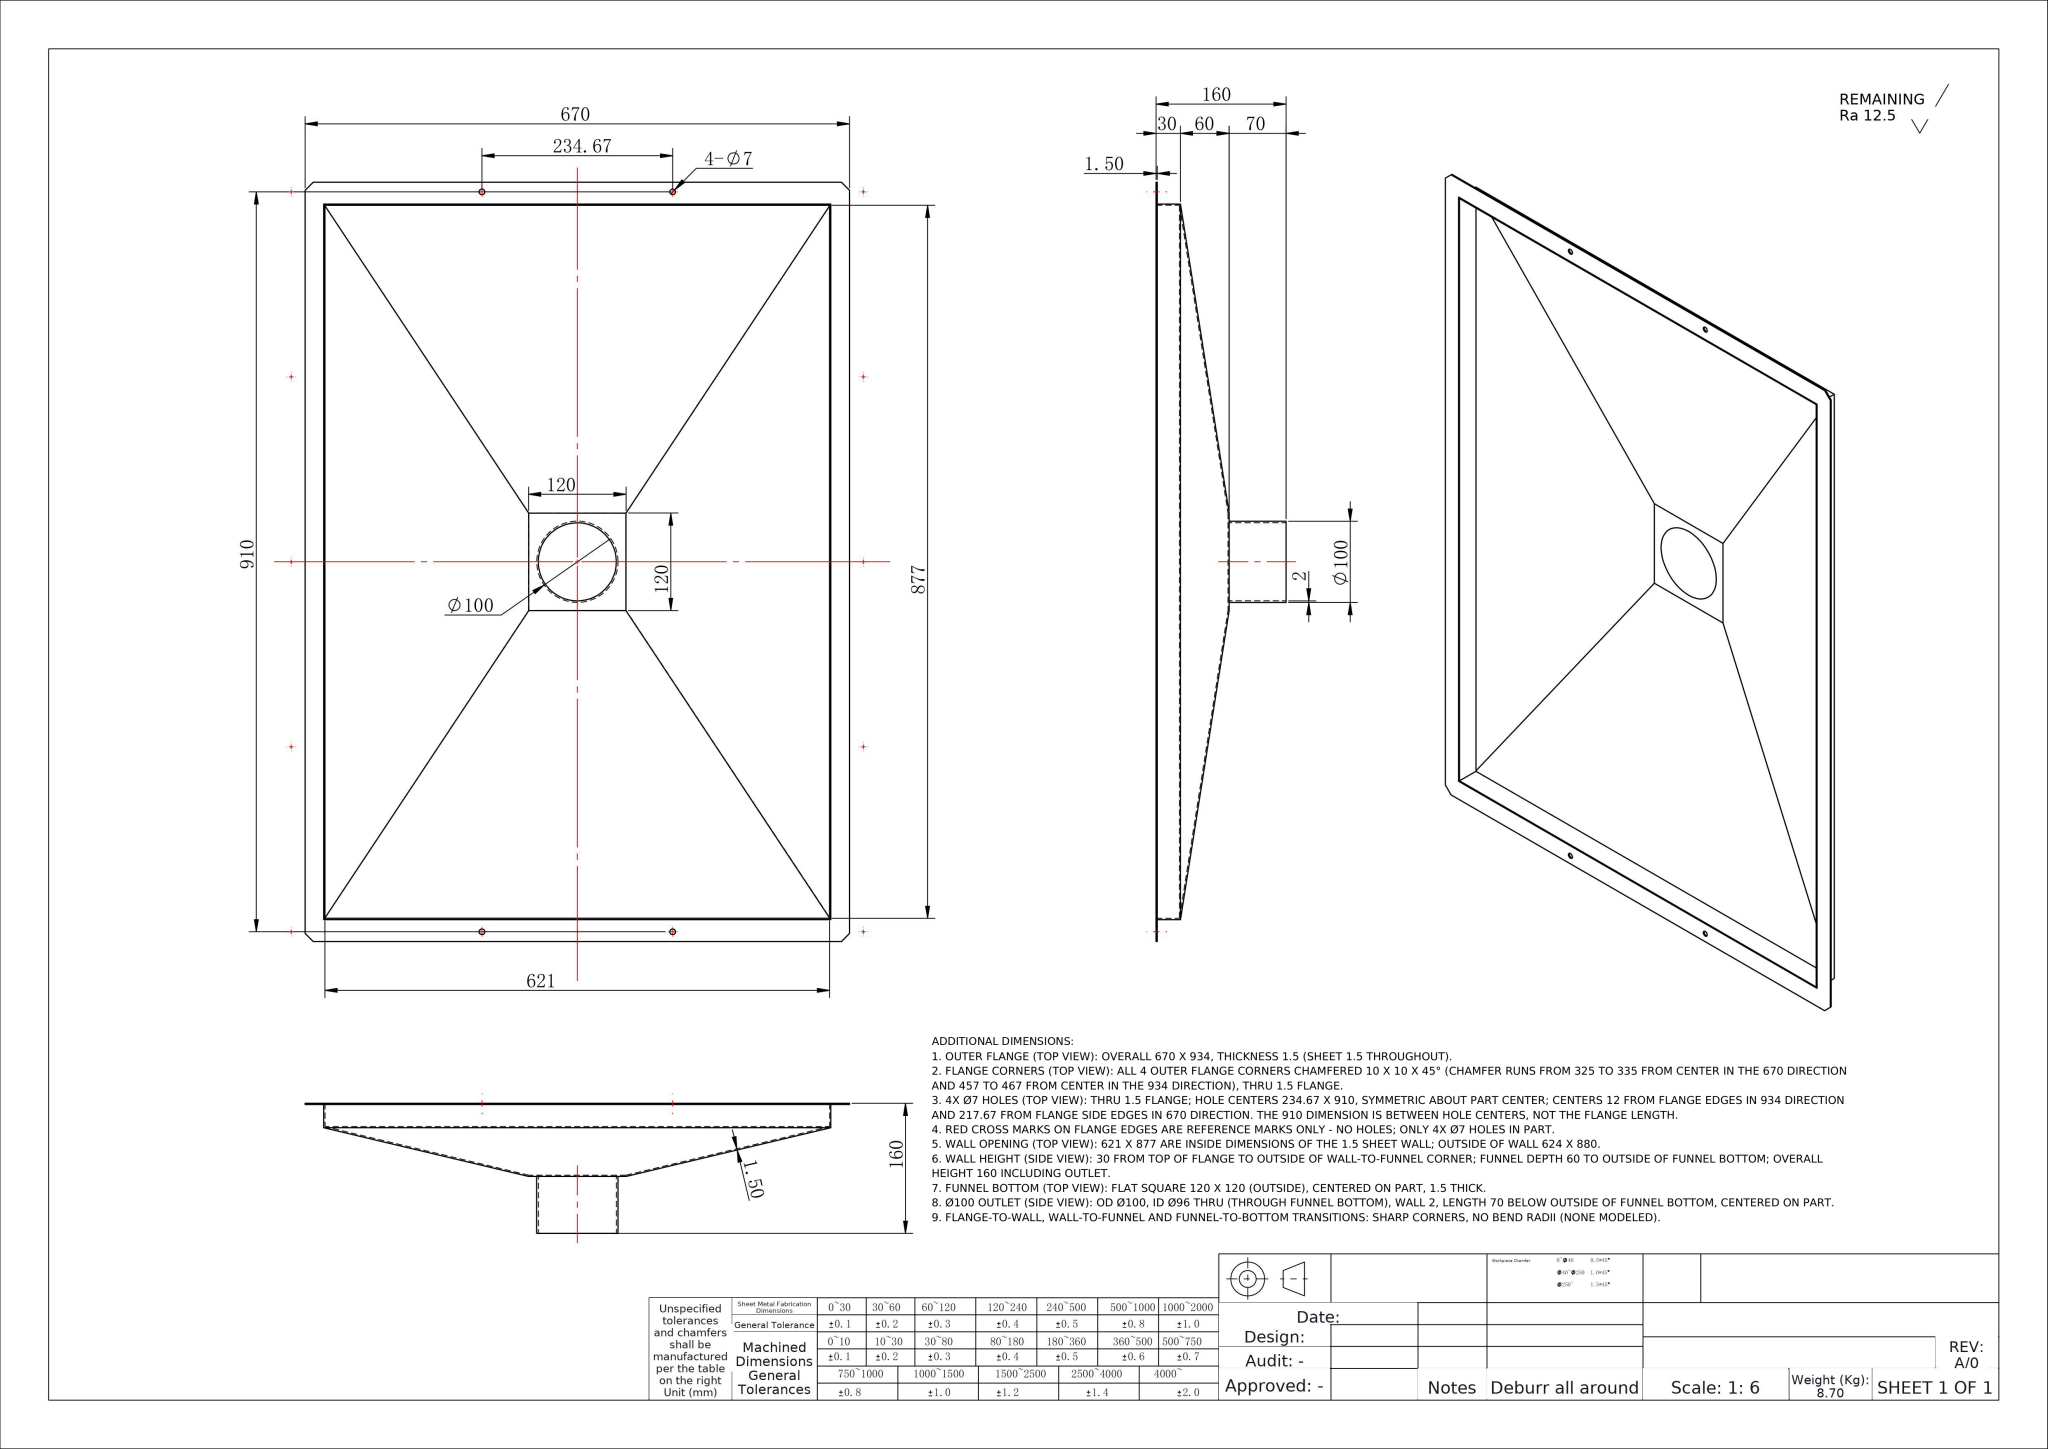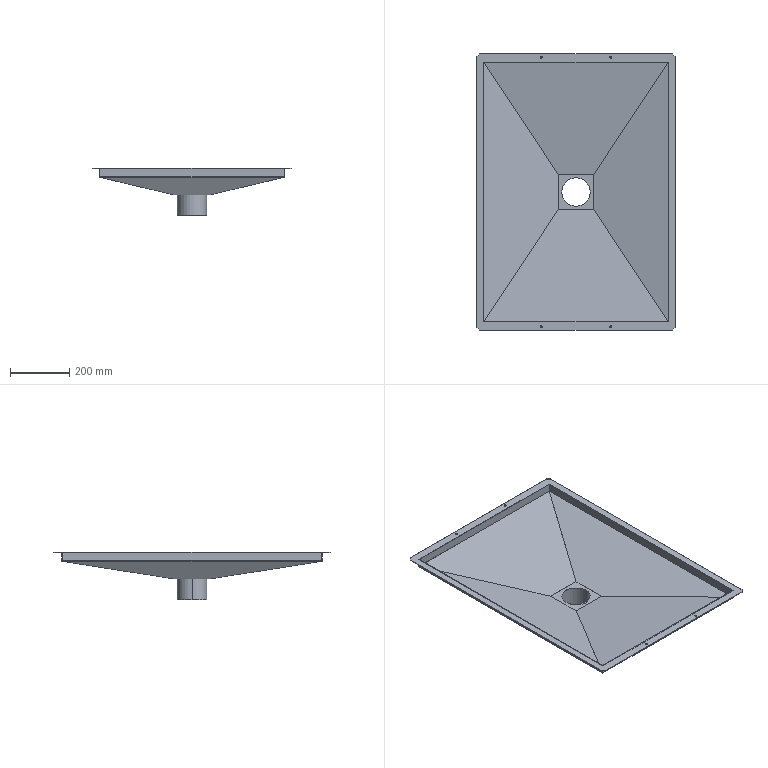Part | NX | mm | 1 solid | 41 faces | box 670 x 934 x 160 mm | volume 1115089 mm3 | plane 29 | cylinder 12 | commonest cylinder face diameters 7 x8 96 x2 100 x2